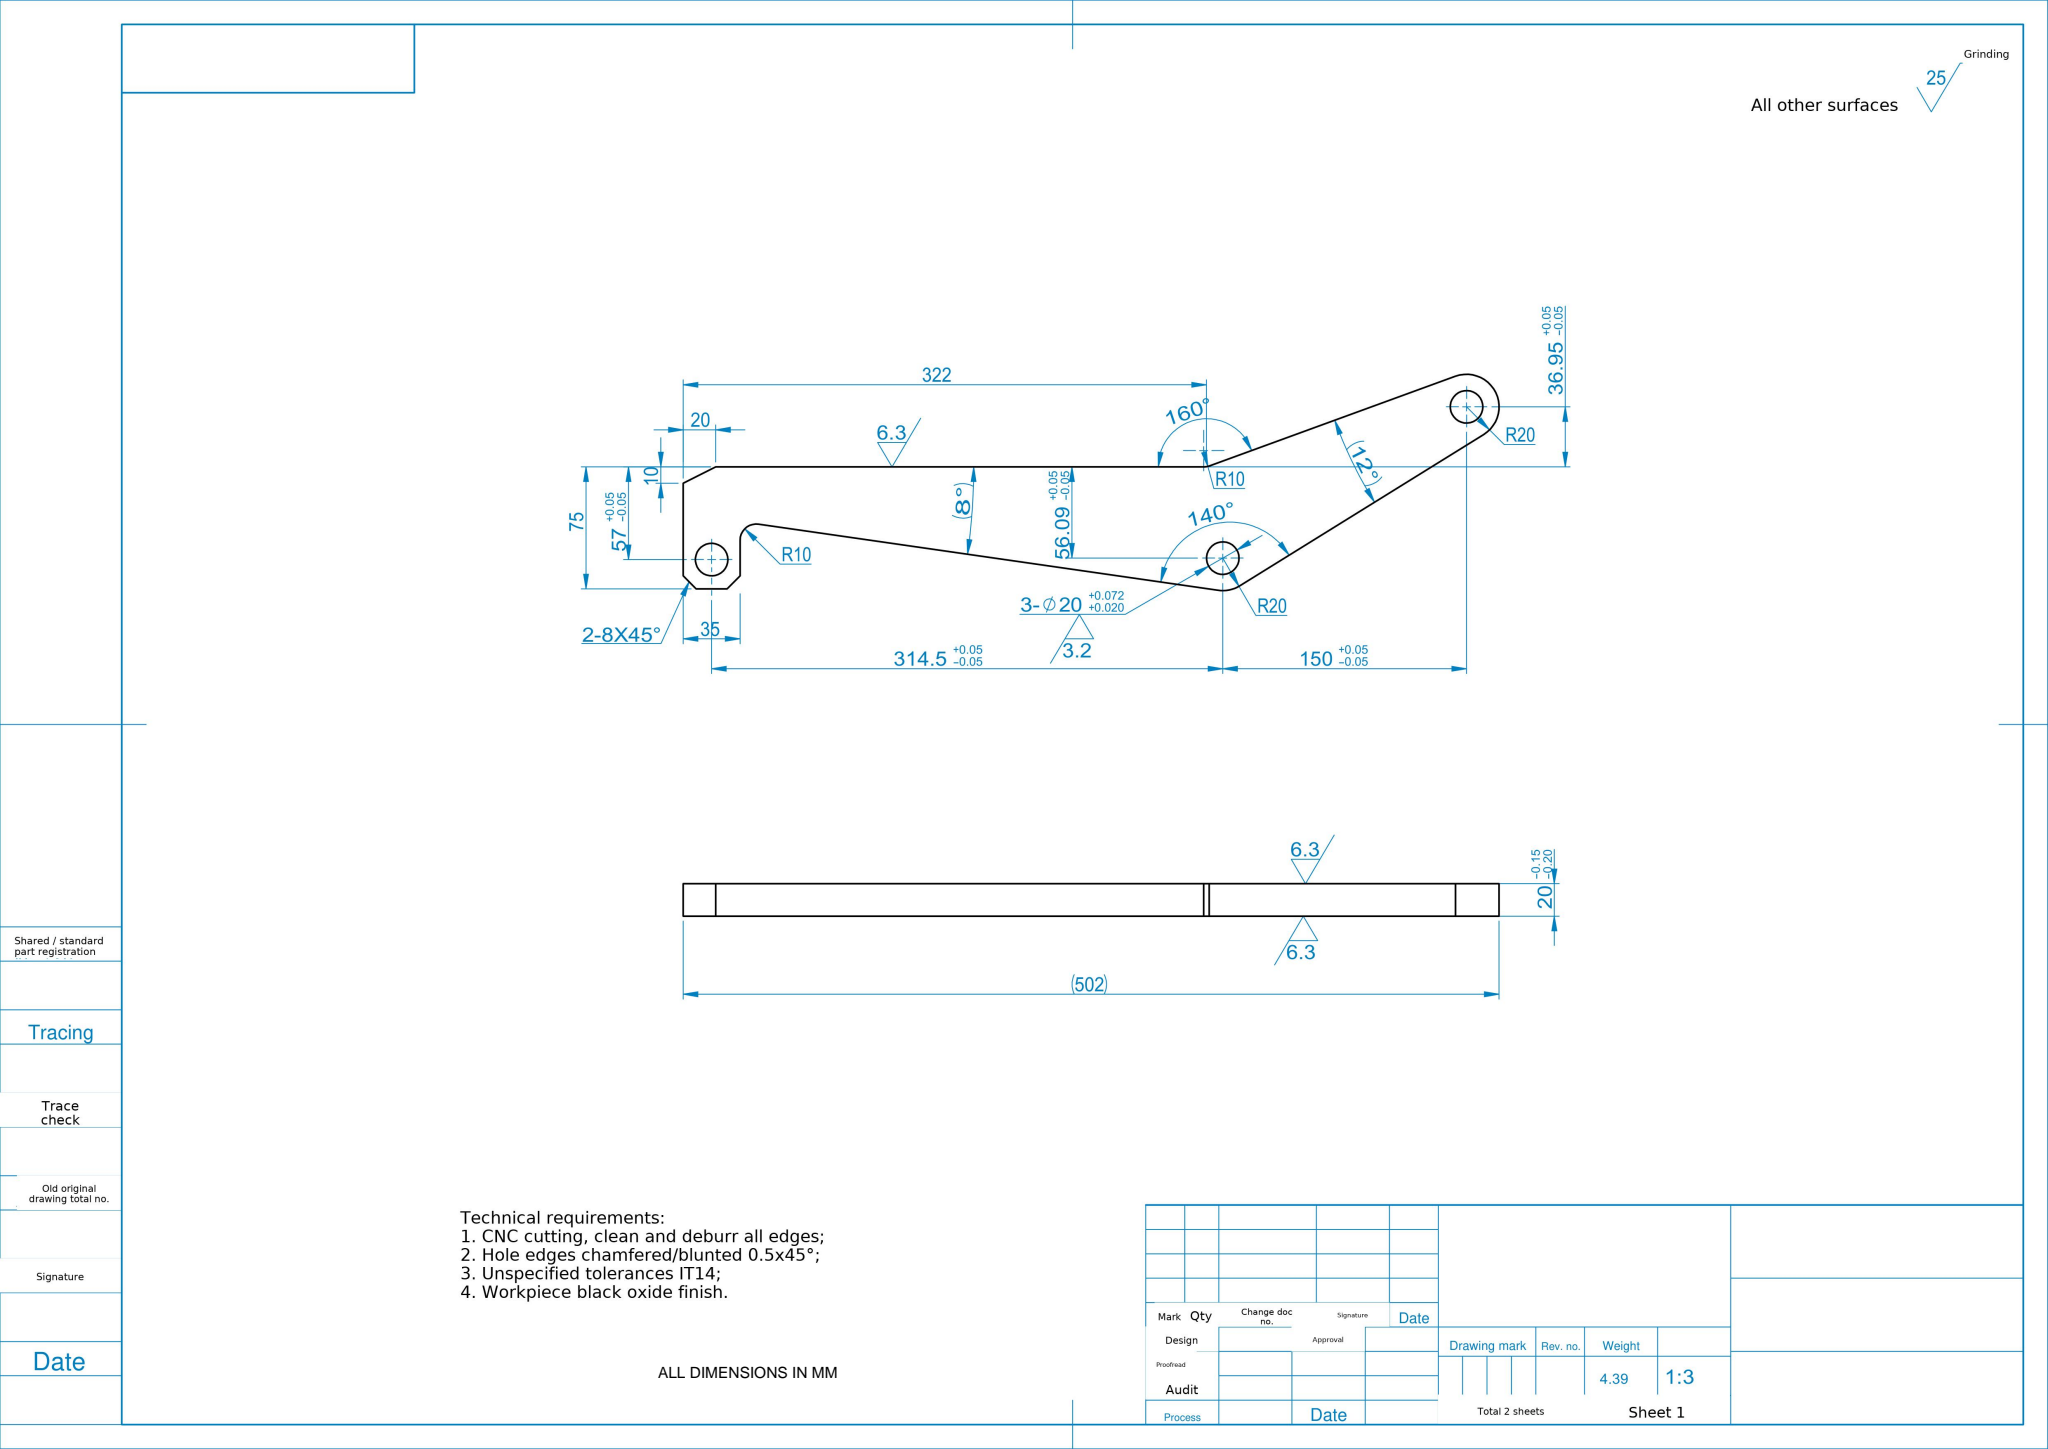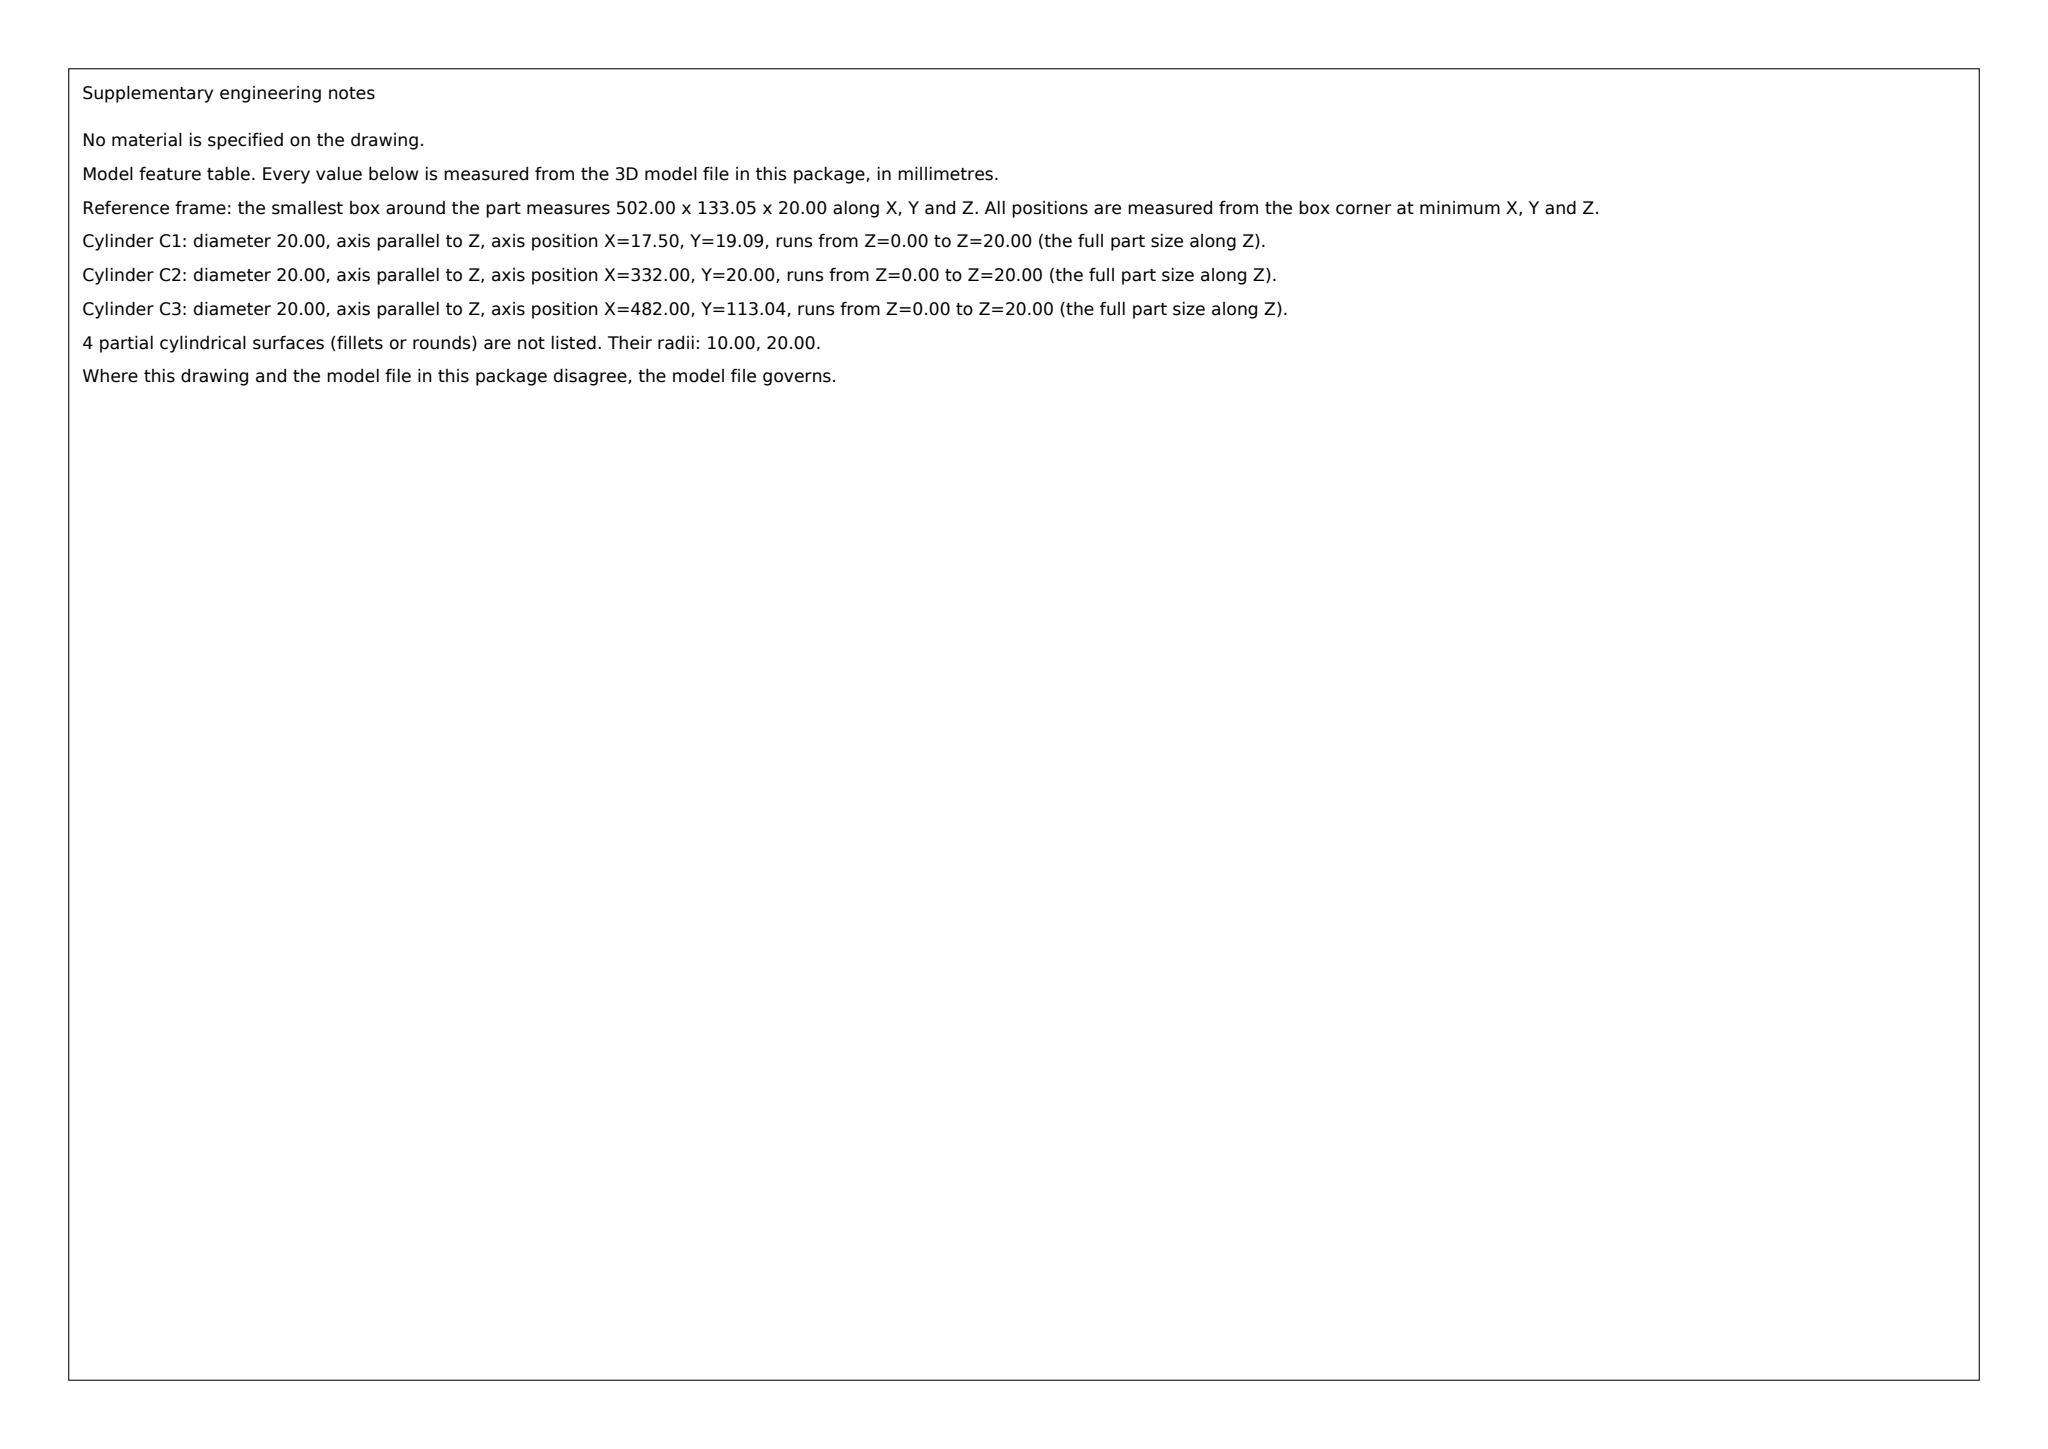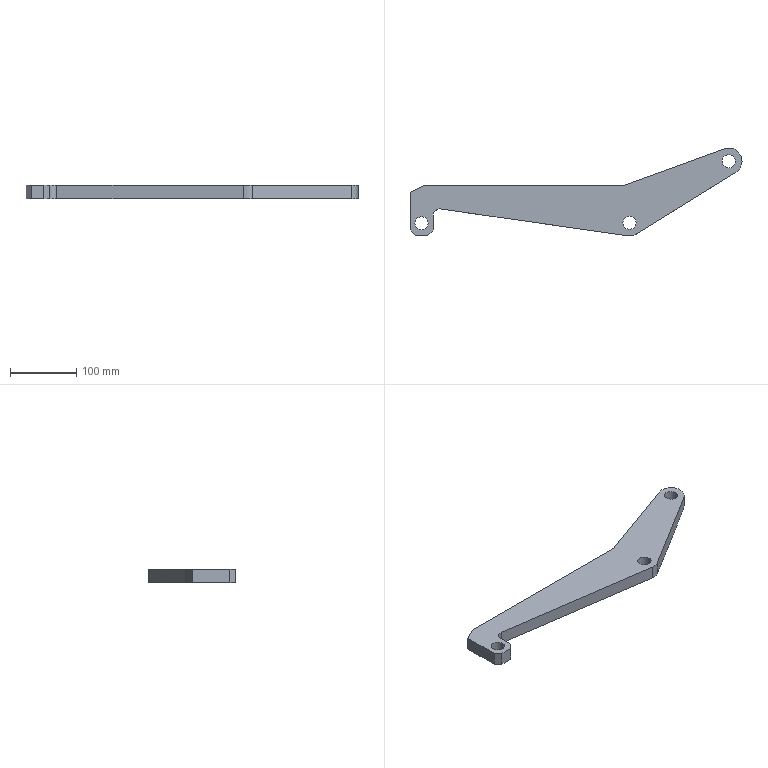Part | SolidWorks | mm | material Plain Carbon Steel | 1 solid | 22 faces | box 502 x 133.05 x 20 mm | volume 562252 mm3 | plane 12 | cylinder 10 | commonest cylinder face diameters 20 x8 40 x2
build123d program:
from build123d import *

# Parameters (mm, degrees)
BOSS_EXTRUDE1_DEPTH = 10
SKETCH2_R           = 10
CUT_EXTRUDE1_DEPTH  = 520.437
CHAMFER2_SIZE       = 8
CHAMFER3_SIZE       = 20
CHAMFER3_SIZE2      = 10
FILLET1_R           = 10
SKETCH5_R           = 10
CUT_EXTRUDE3_DEPTH  = 520.437
SKETCH7_R           = 10
CUT_EXTRUDE5_DEPTH  = 520.437
CUT_EXTRUDE6_DEPTH  = 520.437
FILLET2_R           = 10


with BuildPart() as part:
    # Sketch1 → Boss-Extrude1 (new, symmetric)
    with BuildSketch(Plane.XY):
        with BuildLine():
            Line((322, 75), (475.16, 130.746))
            ThreePointArc((475.16, 130.746), (499.99, 120.689), (492.542, 94.956))
            Line((492.542, 94.956), (342.542, 1.911))
            ThreePointArc((342.542, 1.911), (336.094, -0.6699), (329.151, -0.8894))
            Line((329.151, -0.8894), (45, 40))
            Line((45, 40), (35, 30))
            Line((35, 30), (35, 0))
            Line((35, 0), (0, 0))
            Line((0, 0), (0, 75))
            Line((0, 75), (322, 75))
        make_face()
    extrude(amount=BOSS_EXTRUDE1_DEPTH, both=True)

    # Sketch2 → Cut-Extrude1 (cut, through all)
    with BuildSketch(Plane.XY.offset(10)):
        with Locations((482, 111.952)):
            Circle(SKETCH2_R)
    extrude(amount=-CUT_EXTRUDE1_DEPTH, mode=Mode.SUBTRACT)

    # Chamfer2
    chamfer2_edges = [part.edges().sort_by_distance(p)[0] for p in [
        (35, 0, 0),
        (0, 0, 0),
    ]]
    chamfer(chamfer2_edges, length=CHAMFER2_SIZE)

    # Chamfer3
    chamfer3_edges = [part.edges().sort_by_distance(p)[0] for p in [
        (0, 75, 0),
    ]]
    chamfer3_side = [part.faces().sort_by_distance(p)[0] for p in [
        (161, 75, 0),
    ]]
    chamfer(chamfer3_edges, length=CHAMFER3_SIZE, length2=CHAMFER3_SIZE2, reference=chamfer3_side[0])

    # Fillet1
    fillet1_edges = [part.edges().sort_by_distance(p)[0] for p in [
        (322, 75, 0),
    ]]
    fillet(fillet1_edges, radius=FILLET1_R)

    # Sketch5 → Cut-Extrude3 (cut, through all)
    with BuildSketch(Plane.XY.offset(10)):
        with Locations((17.5, 18)):
            Circle(SKETCH5_R)
    extrude(amount=-CUT_EXTRUDE3_DEPTH, mode=Mode.SUBTRACT)

    # Sketch7 → Cut-Extrude5 (cut, through all)
    with BuildSketch(Plane.XY.offset(10)):
        with Locations((332, 18.907)):
            Circle(SKETCH7_R)
    extrude(amount=-CUT_EXTRUDE5_DEPTH, mode=Mode.SUBTRACT)

    # Sketch8 → Cut-Extrude6 (cut, through all)
    with BuildSketch(Plane.XY.offset(10)):
        Polygon((45, 40), (35, 30), (35, 41.439), align=None)
    extrude(amount=-CUT_EXTRUDE6_DEPTH, mode=Mode.SUBTRACT)

    # Fillet2
    fillet2_edges = [part.edges().sort_by_distance(p)[0] for p in [
        (35, 41.439, 0),
    ]]
    fillet(fillet2_edges, radius=FILLET2_R)


solid = part.part
STEP:
#1=CARTESIAN_POINT('',(322.,18.907,-10.));
#2=VERTEX_POINT('',#1);
#3=CARTESIAN_POINT('',(342.,18.907,-10.));
#4=VERTEX_POINT('',#3);
#5=CARTESIAN_POINT('',(332.,18.907,-10.));
#6=DIRECTION('',(0.,0.,1.));
#7=DIRECTION('',(1.,0.,0.));
#8=AXIS2_PLACEMENT_3D('',#5,#6,#7);
#9=CIRCLE('',#8,10.);
#10=EDGE_CURVE('',#2,#4,#9,.T.);
#11=ORIENTED_EDGE('',*,*,#10,.F.);
#12=CARTESIAN_POINT('',(322.,18.907,10.));
#13=VERTEX_POINT('',#12);
#14=CARTESIAN_POINT('',(322.,18.907,-10.));
#15=DIRECTION('',(0.,0.,1.));
#16=VECTOR('',#15,1000.);
#17=LINE('',#14,#16);
#18=EDGE_CURVE('',#2,#13,#17,.T.);
#19=ORIENTED_EDGE('',*,*,#18,.T.);
#20=CARTESIAN_POINT('',(342.,18.907,10.));
#21=VERTEX_POINT('',#20);
#22=CARTESIAN_POINT('',(332.,18.907,10.));
#23=DIRECTION('',(0.,0.,1.));
#24=DIRECTION('',(1.,0.,0.));
#25=AXIS2_PLACEMENT_3D('',#22,#23,#24);
#26=CIRCLE('',#25,10.);
#27=EDGE_CURVE('',#13,#21,#26,.T.);
#28=ORIENTED_EDGE('',*,*,#27,.T.);
#29=CARTESIAN_POINT('',(342.,18.907,-10.));
#30=DIRECTION('',(0.,0.,1.));
#31=VECTOR('',#30,1000.);
#32=LINE('',#29,#31);
#33=EDGE_CURVE('',#4,#21,#32,.T.);
#34=ORIENTED_EDGE('',*,*,#33,.F.);
#35=EDGE_LOOP('',(#11,#19,#28,#34));
#36=FACE_OUTER_BOUND('',#35,.T.);
#37=CARTESIAN_POINT('',(332.,18.907,-10.));
#38=DIRECTION('',(0.,0.,1.));
#39=DIRECTION('',(1.,0.,0.));
#40=AXIS2_PLACEMENT_3D('',#37,#38,#39);
#41=CYLINDRICAL_SURFACE('',#40,10.);
#42=ADVANCED_FACE('',(#36),#41,.F.);
#43=CARTESIAN_POINT('',(7.5,18.,-10.));
#44=VERTEX_POINT('',#43);
#45=CARTESIAN_POINT('',(27.5,18.,-10.));
#46=VERTEX_POINT('',#45);
#47=CARTESIAN_POINT('',(17.5,18.,-10.));
#48=DIRECTION('',(0.,0.,1.));
#49=DIRECTION('',(1.,0.,0.));
#50=AXIS2_PLACEMENT_3D('',#47,#48,#49);
#51=CIRCLE('',#50,10.);
#52=EDGE_CURVE('',#44,#46,#51,.T.);
#53=ORIENTED_EDGE('',*,*,#52,.F.);
#54=CARTESIAN_POINT('',(7.5,18.,10.));
#55=VERTEX_POINT('',#54);
#56=CARTESIAN_POINT('',(7.5,18.,-10.));
#57=DIRECTION('',(0.,0.,1.));
#58=VECTOR('',#57,1000.);
#59=LINE('',#56,#58);
#60=EDGE_CURVE('',#44,#55,#59,.T.);
#61=ORIENTED_EDGE('',*,*,#60,.T.);
#62=CARTESIAN_POINT('',(27.5,18.,10.));
#63=VERTEX_POINT('',#62);
#64=CARTESIAN_POINT('',(17.5,18.,10.));
#65=DIRECTION('',(0.,0.,1.));
#66=DIRECTION('',(1.,0.,0.));
#67=AXIS2_PLACEMENT_3D('',#64,#65,#66);
#68=CIRCLE('',#67,10.);
#69=EDGE_CURVE('',#55,#63,#68,.T.);
#70=ORIENTED_EDGE('',*,*,#69,.T.);
#71=CARTESIAN_POINT('',(27.5,18.,-10.));
#72=DIRECTION('',(0.,0.,1.));
#73=VECTOR('',#72,1000.);
#74=LINE('',#71,#73);
#75=EDGE_CURVE('',#46,#63,#74,.T.);
#76=ORIENTED_EDGE('',*,*,#75,.F.);
#77=EDGE_LOOP('',(#53,#61,#70,#76));
#78=FACE_OUTER_BOUND('',#77,.T.);
#79=CARTESIAN_POINT('',(17.5,18.,-10.));
#80=DIRECTION('',(0.,0.,1.));
#81=DIRECTION('',(1.,0.,0.));
#82=AXIS2_PLACEMENT_3D('',#79,#80,#81);
#83=CYLINDRICAL_SURFACE('',#82,10.);
#84=ADVANCED_FACE('',(#78),#83,.F.);
#85=CARTESIAN_POINT('',(472.,111.952,-10.));
#86=VERTEX_POINT('',#85);
#87=CARTESIAN_POINT('',(492.,111.952,-10.));
#88=VERTEX_POINT('',#87);
#89=CARTESIAN_POINT('',(482.,111.952,-10.));
#90=DIRECTION('',(0.,0.,1.));
#91=DIRECTION('',(1.,0.,0.));
#92=AXIS2_PLACEMENT_3D('',#89,#90,#91);
#93=CIRCLE('',#92,10.);
#94=EDGE_CURVE('',#86,#88,#93,.T.);
#95=ORIENTED_EDGE('',*,*,#94,.F.);
#96=CARTESIAN_POINT('',(472.,111.952,10.));
#97=VERTEX_POINT('',#96);
#98=CARTESIAN_POINT('',(472.,111.952,-10.));
#99=DIRECTION('',(0.,0.,1.));
#100=VECTOR('',#99,1000.);
#101=LINE('',#98,#100);
#102=EDGE_CURVE('',#86,#97,#101,.T.);
#103=ORIENTED_EDGE('',*,*,#102,.T.);
#104=CARTESIAN_POINT('',(492.,111.952,10.));
#105=VERTEX_POINT('',#104);
#106=CARTESIAN_POINT('',(482.,111.952,10.));
#107=DIRECTION('',(0.,0.,1.));
#108=DIRECTION('',(1.,0.,0.));
#109=AXIS2_PLACEMENT_3D('',#106,#107,#108);
#110=CIRCLE('',#109,10.);
#111=EDGE_CURVE('',#97,#105,#110,.T.);
#112=ORIENTED_EDGE('',*,*,#111,.T.);
#113=CARTESIAN_POINT('',(492.,111.952,-10.));
#114=DIRECTION('',(0.,0.,1.));
#115=VECTOR('',#114,1000.);
#116=LINE('',#113,#115);
#117=EDGE_CURVE('',#88,#105,#116,.T.);
#118=ORIENTED_EDGE('',*,*,#117,.F.);
#119=EDGE_LOOP('',(#95,#103,#112,#118));
#120=FACE_OUTER_BOUND('',#119,.T.);
#121=CARTESIAN_POINT('',(482.,111.952,-10.));
#122=DIRECTION('',(0.,0.,1.));
#123=DIRECTION('',(1.,0.,0.));
#124=AXIS2_PLACEMENT_3D('',#121,#122,#123);
#125=CYLINDRICAL_SURFACE('',#124,10.);
#126=ADVANCED_FACE('',(#120),#125,.F.);
#127=CARTESIAN_POINT('',(46.424,39.795,10.));
#128=VERTEX_POINT('',#127);
#129=CARTESIAN_POINT('',(329.151,-0.8894,10.));
#130=VERTEX_POINT('',#129);
#131=CARTESIAN_POINT('',(45.,40.,10.));
#132=DIRECTION('',(0.9898,-0.1424,0.));
#133=VECTOR('',#132,1000.);
#134=LINE('',#131,#133);
#135=EDGE_CURVE('',#128,#130,#134,.T.);
#136=ORIENTED_EDGE('',*,*,#135,.F.);
#137=CARTESIAN_POINT('',(46.424,39.795,-10.));
#138=VERTEX_POINT('',#137);
#139=CARTESIAN_POINT('',(46.424,39.795,-10.));
#140=DIRECTION('',(0.,0.,-1.));
#141=VECTOR('',#140,1000.);
#142=LINE('',#139,#141);
#143=EDGE_CURVE('',#128,#138,#142,.T.);
#144=ORIENTED_EDGE('',*,*,#143,.T.);
#145=CARTESIAN_POINT('',(329.151,-0.8894,-10.));
#146=VERTEX_POINT('',#145);
#147=CARTESIAN_POINT('',(45.,40.,-10.));
#148=DIRECTION('',(0.9898,-0.1424,0.));
#149=VECTOR('',#148,1000.);
#150=LINE('',#147,#149);
#151=EDGE_CURVE('',#138,#146,#150,.T.);
#152=ORIENTED_EDGE('',*,*,#151,.T.);
#153=CARTESIAN_POINT('',(329.151,-0.8894,10.));
#154=DIRECTION('',(0.,0.,-1.));
#155=VECTOR('',#154,1000.);
#156=LINE('',#153,#155);
#157=EDGE_CURVE('',#130,#146,#156,.T.);
#158=ORIENTED_EDGE('',*,*,#157,.F.);
#159=EDGE_LOOP('',(#136,#144,#152,#158));
#160=FACE_OUTER_BOUND('',#159,.T.);
#161=CARTESIAN_POINT('',(45.,40.,10.));
#162=DIRECTION('',(0.1424,0.9898,0.));
#163=DIRECTION('',(-0.9898,0.1424,0.));
#164=AXIS2_PLACEMENT_3D('',#161,#162,#163);
#165=PLANE('',#164);
#166=ADVANCED_FACE('',(#160),#165,.F.);
#167=CARTESIAN_POINT('',(342.542,1.911,-10.));
#168=VERTEX_POINT('',#167);
#169=CARTESIAN_POINT('',(332.,18.907,-10.));
#170=DIRECTION('',(0.,0.,1.));
#171=DIRECTION('',(1.,0.,0.));
#172=AXIS2_PLACEMENT_3D('',#169,#170,#171);
#173=CIRCLE('',#172,20.);
#174=EDGE_CURVE('',#146,#168,#173,.T.);
#175=ORIENTED_EDGE('',*,*,#174,.T.);
#176=CARTESIAN_POINT('',(342.542,1.911,10.));
#177=VERTEX_POINT('',#176);
#178=CARTESIAN_POINT('',(342.542,1.911,10.));
#179=DIRECTION('',(0.,0.,-1.));
#180=VECTOR('',#179,1000.);
#181=LINE('',#178,#180);
#182=EDGE_CURVE('',#177,#168,#181,.T.);
#183=ORIENTED_EDGE('',*,*,#182,.F.);
#184=CARTESIAN_POINT('',(332.,18.907,10.));
#185=DIRECTION('',(0.,0.,1.));
#186=DIRECTION('',(1.,0.,0.));
#187=AXIS2_PLACEMENT_3D('',#184,#185,#186);
#188=CIRCLE('',#187,20.);
#189=EDGE_CURVE('',#130,#177,#188,.T.);
#190=ORIENTED_EDGE('',*,*,#189,.F.);
#191=ORIENTED_EDGE('',*,*,#157,.T.);
#192=EDGE_LOOP('',(#175,#183,#190,#191));
#193=FACE_OUTER_BOUND('',#192,.T.);
#194=CARTESIAN_POINT('',(332.,18.907,10.));
#195=DIRECTION('',(0.,0.,-1.));
#196=DIRECTION('',(-1.,0.,0.));
#197=AXIS2_PLACEMENT_3D('',#194,#195,#196);
#198=CYLINDRICAL_SURFACE('',#197,20.);
#199=ADVANCED_FACE('',(#193),#198,.T.);
#200=CARTESIAN_POINT('',(492.542,94.956,-10.));
#201=VERTEX_POINT('',#200);
#202=CARTESIAN_POINT('',(342.542,1.911,-10.));
#203=DIRECTION('',(0.8498,0.5271,0.));
#204=VECTOR('',#203,1000.);
#205=LINE('',#202,#204);
#206=EDGE_CURVE('',#168,#201,#205,.T.);
#207=ORIENTED_EDGE('',*,*,#206,.T.);
#208=CARTESIAN_POINT('',(492.542,94.956,10.));
#209=VERTEX_POINT('',#208);
#210=CARTESIAN_POINT('',(492.542,94.956,10.));
#211=DIRECTION('',(0.,0.,-1.));
#212=VECTOR('',#211,1000.);
#213=LINE('',#210,#212);
#214=EDGE_CURVE('',#209,#201,#213,.T.);
#215=ORIENTED_EDGE('',*,*,#214,.F.);
#216=CARTESIAN_POINT('',(342.542,1.911,10.));
#217=DIRECTION('',(0.8498,0.5271,0.));
#218=VECTOR('',#217,1000.);
#219=LINE('',#216,#218);
#220=EDGE_CURVE('',#177,#209,#219,.T.);
#221=ORIENTED_EDGE('',*,*,#220,.F.);
#222=ORIENTED_EDGE('',*,*,#182,.T.);
#223=EDGE_LOOP('',(#207,#215,#221,#222));
#224=FACE_OUTER_BOUND('',#223,.T.);
#225=CARTESIAN_POINT('',(342.542,1.911,10.));
#226=DIRECTION('',(-0.5271,0.8498,0.));
#227=DIRECTION('',(-0.8498,-0.5271,0.));
#228=AXIS2_PLACEMENT_3D('',#225,#226,#227);
#229=PLANE('',#228);
#230=ADVANCED_FACE('',(#224),#229,.F.);
#231=CARTESIAN_POINT('',(475.16,130.746,-10.));
#232=VERTEX_POINT('',#231);
#233=CARTESIAN_POINT('',(482.,111.952,-10.));
#234=DIRECTION('',(0.,0.,1.));
#235=DIRECTION('',(1.,0.,0.));
#236=AXIS2_PLACEMENT_3D('',#233,#234,#235);
#237=CIRCLE('',#236,20.);
#238=EDGE_CURVE('',#201,#232,#237,.T.);
#239=ORIENTED_EDGE('',*,*,#238,.T.);
#240=CARTESIAN_POINT('',(475.16,130.746,10.));
#241=VERTEX_POINT('',#240);
#242=CARTESIAN_POINT('',(475.16,130.746,10.));
#243=DIRECTION('',(0.,0.,-1.));
#244=VECTOR('',#243,1000.);
#245=LINE('',#242,#244);
#246=EDGE_CURVE('',#241,#232,#245,.T.);
#247=ORIENTED_EDGE('',*,*,#246,.F.);
#248=CARTESIAN_POINT('',(482.,111.952,10.));
#249=DIRECTION('',(0.,0.,1.));
#250=DIRECTION('',(1.,0.,0.));
#251=AXIS2_PLACEMENT_3D('',#248,#249,#250);
#252=CIRCLE('',#251,20.);
#253=EDGE_CURVE('',#209,#241,#252,.T.);
#254=ORIENTED_EDGE('',*,*,#253,.F.);
#255=ORIENTED_EDGE('',*,*,#214,.T.);
#256=EDGE_LOOP('',(#239,#247,#254,#255));
#257=FACE_OUTER_BOUND('',#256,.T.);
#258=CARTESIAN_POINT('',(482.,111.952,10.));
#259=DIRECTION('',(0.,0.,-1.));
#260=DIRECTION('',(-1.,0.,0.));
#261=AXIS2_PLACEMENT_3D('',#258,#259,#260);
#262=CYLINDRICAL_SURFACE('',#261,20.);
#263=ADVANCED_FACE('',(#257),#262,.T.);
#264=CARTESIAN_POINT('',(323.657,75.603,-10.));
#265=VERTEX_POINT('',#264);
#266=CARTESIAN_POINT('',(322.,75.,-10.));
#267=DIRECTION('',(-0.9397,-0.342,0.));
#268=VECTOR('',#267,1000.);
#269=LINE('',#266,#268);
#270=EDGE_CURVE('',#232,#265,#269,.T.);
#271=ORIENTED_EDGE('',*,*,#270,.T.);
#272=CARTESIAN_POINT('',(323.657,75.603,10.));
#273=VERTEX_POINT('',#272);
#274=CARTESIAN_POINT('',(323.657,75.603,10.));
#275=DIRECTION('',(0.,0.,1.));
#276=VECTOR('',#275,1000.);
#277=LINE('',#274,#276);
#278=EDGE_CURVE('',#265,#273,#277,.T.);
#279=ORIENTED_EDGE('',*,*,#278,.T.);
#280=CARTESIAN_POINT('',(322.,75.,10.));
#281=DIRECTION('',(-0.9397,-0.342,0.));
#282=VECTOR('',#281,1000.);
#283=LINE('',#280,#282);
#284=EDGE_CURVE('',#241,#273,#283,.T.);
#285=ORIENTED_EDGE('',*,*,#284,.F.);
#286=ORIENTED_EDGE('',*,*,#246,.T.);
#287=EDGE_LOOP('',(#271,#279,#285,#286));
#288=FACE_OUTER_BOUND('',#287,.T.);
#289=CARTESIAN_POINT('',(322.,75.,10.));
#290=DIRECTION('',(0.342,-0.9397,0.));
#291=DIRECTION('',(0.9397,0.342,0.));
#292=AXIS2_PLACEMENT_3D('',#289,#290,#291);
#293=PLANE('',#292);
#294=ADVANCED_FACE('',(#288),#293,.F.);
#295=CARTESIAN_POINT('',(320.237,75.,10.));
#296=VERTEX_POINT('',#295);
#297=CARTESIAN_POINT('',(20.,75.,10.));
#298=VERTEX_POINT('',#297);
#299=CARTESIAN_POINT('',(0.,75.,10.));
#300=DIRECTION('',(-1.,-0.,0.));
#301=VECTOR('',#300,1000.);
#302=LINE('',#299,#301);
#303=EDGE_CURVE('',#296,#298,#302,.T.);
#304=ORIENTED_EDGE('',*,*,#303,.F.);
#305=CARTESIAN_POINT('',(320.237,75.,-10.));
#306=VERTEX_POINT('',#305);
#307=CARTESIAN_POINT('',(320.237,75.,-10.));
#308=DIRECTION('',(0.,0.,-1.));
#309=VECTOR('',#308,1000.);
#310=LINE('',#307,#309);
#311=EDGE_CURVE('',#296,#306,#310,.T.);
#312=ORIENTED_EDGE('',*,*,#311,.T.);
#313=CARTESIAN_POINT('',(20.,75.,-10.));
#314=VERTEX_POINT('',#313);
#315=CARTESIAN_POINT('',(0.,75.,-10.));
#316=DIRECTION('',(-1.,-0.,0.));
#317=VECTOR('',#316,1000.);
#318=LINE('',#315,#317);
#319=EDGE_CURVE('',#306,#314,#318,.T.);
#320=ORIENTED_EDGE('',*,*,#319,.T.);
#321=CARTESIAN_POINT('',(20.,75.,10.));
#322=DIRECTION('',(0.,0.,1.));
#323=VECTOR('',#322,1000.);
#324=LINE('',#321,#323);
#325=EDGE_CURVE('',#314,#298,#324,.T.);
#326=ORIENTED_EDGE('',*,*,#325,.T.);
#327=EDGE_LOOP('',(#304,#312,#320,#326));
#328=FACE_OUTER_BOUND('',#327,.T.);
#329=CARTESIAN_POINT('',(0.,75.,10.));
#330=DIRECTION('',(0.,-1.,0.));
#331=DIRECTION('',(1.,0.,0.));
#332=AXIS2_PLACEMENT_3D('',#329,#330,#331);
#333=PLANE('',#332);
#334=ADVANCED_FACE('',(#328),#333,.F.);
#335=CARTESIAN_POINT('',(-0.,65.,10.));
#336=VERTEX_POINT('',#335);
#337=CARTESIAN_POINT('',(-0.,8.,10.));
#338=VERTEX_POINT('',#337);
#339=CARTESIAN_POINT('',(0.,0.,10.));
#340=DIRECTION('',(0.,-1.,0.));
#341=VECTOR('',#340,1000.);
#342=LINE('',#339,#341);
#343=EDGE_CURVE('',#336,#338,#342,.T.);
#344=ORIENTED_EDGE('',*,*,#343,.F.);
#345=CARTESIAN_POINT('',(-0.,65.,-10.));
#346=VERTEX_POINT('',#345);
#347=CARTESIAN_POINT('',(0.,65.,10.));
#348=DIRECTION('',(0.,0.,-1.));
#349=VECTOR('',#348,1000.);
#350=LINE('',#347,#349);
#351=EDGE_CURVE('',#336,#346,#350,.T.);
#352=ORIENTED_EDGE('',*,*,#351,.T.);
#353=CARTESIAN_POINT('',(0.,8.,-10.));
#354=VERTEX_POINT('',#353);
#355=CARTESIAN_POINT('',(0.,0.,-10.));
#356=DIRECTION('',(0.,-1.,0.));
#357=VECTOR('',#356,1000.);
#358=LINE('',#355,#357);
#359=EDGE_CURVE('',#346,#354,#358,.T.);
#360=ORIENTED_EDGE('',*,*,#359,.T.);
#361=CARTESIAN_POINT('',(0.,8.,10.));
#362=DIRECTION('',(0.,0.,1.));
#363=VECTOR('',#362,1000.);
#364=LINE('',#361,#363);
#365=EDGE_CURVE('',#354,#338,#364,.T.);
#366=ORIENTED_EDGE('',*,*,#365,.T.);
#367=EDGE_LOOP('',(#344,#352,#360,#366));
#368=FACE_OUTER_BOUND('',#367,.T.);
#369=CARTESIAN_POINT('',(0.,0.,10.));
#370=DIRECTION('',(1.,0.,0.));
#371=DIRECTION('',(0.,0.,-1.));
#372=AXIS2_PLACEMENT_3D('',#369,#370,#371);
#373=PLANE('',#372);
#374=ADVANCED_FACE('',(#368),#373,.F.);
#375=CARTESIAN_POINT('',(8.,-0.,-10.));
#376=VERTEX_POINT('',#375);
#377=CARTESIAN_POINT('',(27.,0.,-10.));
#378=VERTEX_POINT('',#377);
#379=CARTESIAN_POINT('',(35.,0.,-10.));
#380=DIRECTION('',(1.,0.,0.));
#381=VECTOR('',#380,1000.);
#382=LINE('',#379,#381);
#383=EDGE_CURVE('',#376,#378,#382,.T.);
#384=ORIENTED_EDGE('',*,*,#383,.T.);
#385=CARTESIAN_POINT('',(27.,-0.,10.));
#386=VERTEX_POINT('',#385);
#387=CARTESIAN_POINT('',(27.,0.,10.));
#388=DIRECTION('',(0.,0.,1.));
#389=VECTOR('',#388,1000.);
#390=LINE('',#387,#389);
#391=EDGE_CURVE('',#378,#386,#390,.T.);
#392=ORIENTED_EDGE('',*,*,#391,.T.);
#393=CARTESIAN_POINT('',(8.,0.,10.));
#394=VERTEX_POINT('',#393);
#395=CARTESIAN_POINT('',(35.,0.,10.));
#396=DIRECTION('',(1.,0.,0.));
#397=VECTOR('',#396,1000.);
#398=LINE('',#395,#397);
#399=EDGE_CURVE('',#394,#386,#398,.T.);
#400=ORIENTED_EDGE('',*,*,#399,.F.);
#401=CARTESIAN_POINT('',(8.,0.,10.));
#402=DIRECTION('',(0.,0.,-1.));
#403=VECTOR('',#402,1000.);
#404=LINE('',#401,#403);
#405=EDGE_CURVE('',#394,#376,#404,.T.);
#406=ORIENTED_EDGE('',*,*,#405,.T.);
#407=EDGE_LOOP('',(#384,#392,#400,#406));
#408=FACE_OUTER_BOUND('',#407,.T.);
#409=CARTESIAN_POINT('',(35.,0.,10.));
#410=DIRECTION('',(-0.,1.,0.));
#411=DIRECTION('',(-1.,-0.,0.));
#412=AXIS2_PLACEMENT_3D('',#409,#410,#411);
#413=PLANE('',#412);
#414=ADVANCED_FACE('',(#408),#413,.F.);
#415=CARTESIAN_POINT('',(35.,8.,-10.));
#416=VERTEX_POINT('',#415);
#417=CARTESIAN_POINT('',(35.,29.897,-10.));
#418=VERTEX_POINT('',#417);
#419=CARTESIAN_POINT('',(35.,30.,-10.));
#420=DIRECTION('',(0.,1.,0.));
#421=VECTOR('',#420,1000.);
#422=LINE('',#419,#421);
#423=EDGE_CURVE('',#416,#418,#422,.T.);
#424=ORIENTED_EDGE('',*,*,#423,.T.);
#425=CARTESIAN_POINT('',(35.,29.897,10.));
#426=VERTEX_POINT('',#425);
#427=CARTESIAN_POINT('',(35.,29.897,10.));
#428=DIRECTION('',(0.,0.,1.));
#429=VECTOR('',#428,1000.);
#430=LINE('',#427,#429);
#431=EDGE_CURVE('',#418,#426,#430,.T.);
#432=ORIENTED_EDGE('',*,*,#431,.T.);
#433=CARTESIAN_POINT('',(35.,8.,10.));
#434=VERTEX_POINT('',#433);
#435=CARTESIAN_POINT('',(35.,30.,10.));
#436=DIRECTION('',(0.,1.,0.));
#437=VECTOR('',#436,1000.);
#438=LINE('',#435,#437);
#439=EDGE_CURVE('',#434,#426,#438,.T.);
#440=ORIENTED_EDGE('',*,*,#439,.F.);
#441=CARTESIAN_POINT('',(35.,8.,10.));
#442=DIRECTION('',(0.,0.,-1.));
#443=VECTOR('',#442,1000.);
#444=LINE('',#441,#443);
#445=EDGE_CURVE('',#434,#416,#444,.T.);
#446=ORIENTED_EDGE('',*,*,#445,.T.);
#447=EDGE_LOOP('',(#424,#432,#440,#446));
#448=FACE_OUTER_BOUND('',#447,.T.);
#449=CARTESIAN_POINT('',(35.,30.,10.));
#450=DIRECTION('',(-1.,0.,0.));
#451=DIRECTION('',(0.,0.,1.));
#452=AXIS2_PLACEMENT_3D('',#449,#450,#451);
#453=PLANE('',#452);
#454=ADVANCED_FACE('',(#448),#453,.F.);
#455=ORIENTED_EDGE('',*,*,#439,.T.);
#456=CARTESIAN_POINT('',(45.,29.897,10.));
#457=DIRECTION('',(0.,0.,-1.));
#458=DIRECTION('',(1.,0.,0.));
#459=AXIS2_PLACEMENT_3D('',#456,#457,#458);
#460=CIRCLE('',#459,10.);
#461=EDGE_CURVE('',#426,#128,#460,.T.);
#462=ORIENTED_EDGE('',*,*,#461,.T.);
#463=ORIENTED_EDGE('',*,*,#135,.T.);
#464=ORIENTED_EDGE('',*,*,#189,.T.);
#465=ORIENTED_EDGE('',*,*,#220,.T.);
#466=ORIENTED_EDGE('',*,*,#253,.T.);
#467=ORIENTED_EDGE('',*,*,#284,.T.);
#468=CARTESIAN_POINT('',(320.237,85.,10.));
#469=DIRECTION('',(0.,0.,-1.));
#470=DIRECTION('',(1.,0.,0.));
#471=AXIS2_PLACEMENT_3D('',#468,#469,#470);
#472=CIRCLE('',#471,10.);
#473=EDGE_CURVE('',#273,#296,#472,.T.);
#474=ORIENTED_EDGE('',*,*,#473,.T.);
#475=ORIENTED_EDGE('',*,*,#303,.T.);
#476=CARTESIAN_POINT('',(247.163,188.581,10.));
#477=DIRECTION('',(-0.8944,-0.4472,0.));
#478=VECTOR('',#477,1000.);
#479=LINE('',#476,#478);
#480=EDGE_CURVE('',#298,#336,#479,.T.);
#481=ORIENTED_EDGE('',*,*,#480,.T.);
#482=ORIENTED_EDGE('',*,*,#343,.T.);
#483=CARTESIAN_POINT('',(160.547,-152.547,10.));
#484=DIRECTION('',(0.7071,-0.7071,0.));
#485=VECTOR('',#484,1000.);
#486=LINE('',#483,#485);
#487=EDGE_CURVE('',#338,#394,#486,.T.);
#488=ORIENTED_EDGE('',*,*,#487,.T.);
#489=ORIENTED_EDGE('',*,*,#399,.T.);
#490=CARTESIAN_POINT('',(188.953,161.953,10.));
#491=DIRECTION('',(0.7071,0.7071,0.));
#492=VECTOR('',#491,1000.);
#493=LINE('',#490,#492);
#494=EDGE_CURVE('',#386,#434,#493,.T.);
#495=ORIENTED_EDGE('',*,*,#494,.T.);
#496=EDGE_LOOP('',(#455,#462,#463,#464,#465,#466,#467,#474,#475,#481,#482,#488,#489,#495));
#497=FACE_OUTER_BOUND('',#496,.T.);
#498=CARTESIAN_POINT('',(332.,18.907,10.));
#499=DIRECTION('',(0.,0.,1.));
#500=DIRECTION('',(1.,0.,0.));
#501=AXIS2_PLACEMENT_3D('',#498,#499,#500);
#502=CIRCLE('',#501,10.);
#503=EDGE_CURVE('',#21,#13,#502,.T.);
#504=ORIENTED_EDGE('',*,*,#503,.F.);
#505=ORIENTED_EDGE('',*,*,#27,.F.);
#506=EDGE_LOOP('',(#504,#505));
#507=FACE_BOUND('',#506,.T.);
#508=CARTESIAN_POINT('',(17.5,18.,10.));
#509=DIRECTION('',(0.,0.,1.));
#510=DIRECTION('',(1.,0.,0.));
#511=AXIS2_PLACEMENT_3D('',#508,#509,#510);
#512=CIRCLE('',#511,10.);
#513=EDGE_CURVE('',#63,#55,#512,.T.);
#514=ORIENTED_EDGE('',*,*,#513,.F.);
#515=ORIENTED_EDGE('',*,*,#69,.F.);
#516=EDGE_LOOP('',(#514,#515));
#517=FACE_BOUND('',#516,.T.);
#518=CARTESIAN_POINT('',(482.,111.952,10.));
#519=DIRECTION('',(0.,0.,1.));
#520=DIRECTION('',(1.,0.,0.));
#521=AXIS2_PLACEMENT_3D('',#518,#519,#520);
#522=CIRCLE('',#521,10.);
#523=EDGE_CURVE('',#105,#97,#522,.T.);
#524=ORIENTED_EDGE('',*,*,#523,.F.);
#525=ORIENTED_EDGE('',*,*,#111,.F.);
#526=EDGE_LOOP('',(#524,#525));
#527=FACE_BOUND('',#526,.T.);
#528=CARTESIAN_POINT('',(332.,18.907,10.));
#529=DIRECTION('',(0.,0.,1.));
#530=DIRECTION('',(1.,0.,0.));
#531=AXIS2_PLACEMENT_3D('',#528,#529,#530);
#532=PLANE('',#531);
#533=ADVANCED_FACE('',(#497,#507,#517,#527),#532,.T.);
#534=CARTESIAN_POINT('',(332.,18.907,-10.));
#535=DIRECTION('',(0.,0.,1.));
#536=DIRECTION('',(1.,0.,0.));
#537=AXIS2_PLACEMENT_3D('',#534,#535,#536);
#538=CIRCLE('',#537,10.);
#539=EDGE_CURVE('',#4,#2,#538,.T.);
#540=ORIENTED_EDGE('',*,*,#539,.T.);
#541=ORIENTED_EDGE('',*,*,#10,.T.);
#542=EDGE_LOOP('',(#540,#541));
#543=FACE_BOUND('',#542,.T.);
#544=CARTESIAN_POINT('',(17.5,18.,-10.));
#545=DIRECTION('',(0.,0.,1.));
#546=DIRECTION('',(1.,0.,0.));
#547=AXIS2_PLACEMENT_3D('',#544,#545,#546);
#548=CIRCLE('',#547,10.);
#549=EDGE_CURVE('',#46,#44,#548,.T.);
#550=ORIENTED_EDGE('',*,*,#549,.T.);
#551=ORIENTED_EDGE('',*,*,#52,.T.);
#552=EDGE_LOOP('',(#550,#551));
#553=FACE_BOUND('',#552,.T.);
#554=CARTESIAN_POINT('',(482.,111.952,-10.));
#555=DIRECTION('',(0.,0.,1.));
#556=DIRECTION('',(1.,0.,0.));
#557=AXIS2_PLACEMENT_3D('',#554,#555,#556);
#558=CIRCLE('',#557,10.);
#559=EDGE_CURVE('',#88,#86,#558,.T.);
#560=ORIENTED_EDGE('',*,*,#559,.T.);
#561=ORIENTED_EDGE('',*,*,#94,.T.);
#562=EDGE_LOOP('',(#560,#561));
#563=FACE_BOUND('',#562,.T.);
#564=ORIENTED_EDGE('',*,*,#151,.F.);
#565=CARTESIAN_POINT('',(45.,29.897,-10.));
#566=DIRECTION('',(0.,0.,1.));
#567=DIRECTION('',(1.,0.,0.));
#568=AXIS2_PLACEMENT_3D('',#565,#566,#567);
#569=CIRCLE('',#568,10.);
#570=EDGE_CURVE('',#138,#418,#569,.T.);
#571=ORIENTED_EDGE('',*,*,#570,.T.);
#572=ORIENTED_EDGE('',*,*,#423,.F.);
#573=CARTESIAN_POINT('',(35.,8.,-10.));
#574=DIRECTION('',(-0.7071,-0.7071,0.));
#575=VECTOR('',#574,1000.);
#576=LINE('',#573,#575);
#577=EDGE_CURVE('',#416,#378,#576,.T.);
#578=ORIENTED_EDGE('',*,*,#577,.T.);
#579=ORIENTED_EDGE('',*,*,#383,.F.);
#580=CARTESIAN_POINT('',(8.,0.,-10.));
#581=DIRECTION('',(-0.7071,0.7071,0.));
#582=VECTOR('',#581,1000.);
#583=LINE('',#580,#582);
#584=EDGE_CURVE('',#376,#354,#583,.T.);
#585=ORIENTED_EDGE('',*,*,#584,.T.);
#586=ORIENTED_EDGE('',*,*,#359,.F.);
#587=CARTESIAN_POINT('',(0.,65.,-10.));
#588=DIRECTION('',(0.8944,0.4472,0.));
#589=VECTOR('',#588,1000.);
#590=LINE('',#587,#589);
#591=EDGE_CURVE('',#346,#314,#590,.T.);
#592=ORIENTED_EDGE('',*,*,#591,.T.);
#593=ORIENTED_EDGE('',*,*,#319,.F.);
#594=CARTESIAN_POINT('',(320.237,85.,-10.));
#595=DIRECTION('',(0.,0.,1.));
#596=DIRECTION('',(1.,0.,0.));
#597=AXIS2_PLACEMENT_3D('',#594,#595,#596);
#598=CIRCLE('',#597,10.);
#599=EDGE_CURVE('',#306,#265,#598,.T.);
#600=ORIENTED_EDGE('',*,*,#599,.T.);
#601=ORIENTED_EDGE('',*,*,#270,.F.);
#602=ORIENTED_EDGE('',*,*,#238,.F.);
#603=ORIENTED_EDGE('',*,*,#206,.F.);
#604=ORIENTED_EDGE('',*,*,#174,.F.);
#605=EDGE_LOOP('',(#564,#571,#572,#578,#579,#585,#586,#592,#593,#600,#601,#602,#603,#604));
#606=FACE_OUTER_BOUND('',#605,.T.);
#607=CARTESIAN_POINT('',(332.,18.907,-10.));
#608=DIRECTION('',(0.,0.,1.));
#609=DIRECTION('',(1.,0.,0.));
#610=AXIS2_PLACEMENT_3D('',#607,#608,#609);
#611=PLANE('',#610);
#612=ADVANCED_FACE('',(#543,#553,#563,#606),#611,.F.);
#613=ORIENTED_EDGE('',*,*,#102,.F.);
#614=ORIENTED_EDGE('',*,*,#559,.F.);
#615=ORIENTED_EDGE('',*,*,#117,.T.);
#616=ORIENTED_EDGE('',*,*,#523,.T.);
#617=EDGE_LOOP('',(#613,#614,#615,#616));
#618=FACE_OUTER_BOUND('',#617,.T.);
#619=CARTESIAN_POINT('',(482.,111.952,-10.));
#620=DIRECTION('',(0.,0.,1.));
#621=DIRECTION('',(1.,0.,0.));
#622=AXIS2_PLACEMENT_3D('',#619,#620,#621);
#623=CYLINDRICAL_SURFACE('',#622,10.);
#624=ADVANCED_FACE('',(#618),#623,.F.);
#625=ORIENTED_EDGE('',*,*,#494,.F.);
#626=ORIENTED_EDGE('',*,*,#391,.F.);
#627=ORIENTED_EDGE('',*,*,#577,.F.);
#628=ORIENTED_EDGE('',*,*,#445,.F.);
#629=EDGE_LOOP('',(#625,#626,#627,#628));
#630=FACE_OUTER_BOUND('',#629,.T.);
#631=CARTESIAN_POINT('',(35.,8.,10.));
#632=DIRECTION('',(-0.7071,0.7071,0.));
#633=DIRECTION('',(0.,0.,-1.));
#634=AXIS2_PLACEMENT_3D('',#631,#632,#633);
#635=PLANE('',#634);
#636=ADVANCED_FACE('',(#630),#635,.F.);
#637=ORIENTED_EDGE('',*,*,#487,.F.);
#638=ORIENTED_EDGE('',*,*,#365,.F.);
#639=ORIENTED_EDGE('',*,*,#584,.F.);
#640=ORIENTED_EDGE('',*,*,#405,.F.);
#641=EDGE_LOOP('',(#637,#638,#639,#640));
#642=FACE_OUTER_BOUND('',#641,.T.);
#643=CARTESIAN_POINT('',(8.,0.,10.));
#644=DIRECTION('',(0.7071,0.7071,0.));
#645=DIRECTION('',(0.,0.,-1.));
#646=AXIS2_PLACEMENT_3D('',#643,#644,#645);
#647=PLANE('',#646);
#648=ADVANCED_FACE('',(#642),#647,.F.);
#649=ORIENTED_EDGE('',*,*,#480,.F.);
#650=ORIENTED_EDGE('',*,*,#325,.F.);
#651=ORIENTED_EDGE('',*,*,#591,.F.);
#652=ORIENTED_EDGE('',*,*,#351,.F.);
#653=EDGE_LOOP('',(#649,#650,#651,#652));
#654=FACE_OUTER_BOUND('',#653,.T.);
#655=CARTESIAN_POINT('',(0.,65.,10.));
#656=DIRECTION('',(0.4472,-0.8944,0.));
#657=DIRECTION('',(0.,0.,-1.));
#658=AXIS2_PLACEMENT_3D('',#655,#656,#657);
#659=PLANE('',#658);
#660=ADVANCED_FACE('',(#654),#659,.F.);
#661=ORIENTED_EDGE('',*,*,#473,.F.);
#662=ORIENTED_EDGE('',*,*,#278,.F.);
#663=ORIENTED_EDGE('',*,*,#599,.F.);
#664=ORIENTED_EDGE('',*,*,#311,.F.);
#665=EDGE_LOOP('',(#661,#662,#663,#664));
#666=FACE_OUTER_BOUND('',#665,.T.);
#667=CARTESIAN_POINT('',(320.237,85.,10.));
#668=DIRECTION('',(0.,0.,1.));
#669=DIRECTION('',(1.,0.,0.));
#670=AXIS2_PLACEMENT_3D('',#667,#668,#669);
#671=CYLINDRICAL_SURFACE('',#670,10.);
#672=ADVANCED_FACE('',(#666),#671,.F.);
#673=ORIENTED_EDGE('',*,*,#60,.F.);
#674=ORIENTED_EDGE('',*,*,#549,.F.);
#675=ORIENTED_EDGE('',*,*,#75,.T.);
#676=ORIENTED_EDGE('',*,*,#513,.T.);
#677=EDGE_LOOP('',(#673,#674,#675,#676));
#678=FACE_OUTER_BOUND('',#677,.T.);
#679=CARTESIAN_POINT('',(17.5,18.,-10.));
#680=DIRECTION('',(0.,0.,1.));
#681=DIRECTION('',(1.,0.,0.));
#682=AXIS2_PLACEMENT_3D('',#679,#680,#681);
#683=CYLINDRICAL_SURFACE('',#682,10.);
#684=ADVANCED_FACE('',(#678),#683,.F.);
#685=ORIENTED_EDGE('',*,*,#18,.F.);
#686=ORIENTED_EDGE('',*,*,#539,.F.);
#687=ORIENTED_EDGE('',*,*,#33,.T.);
#688=ORIENTED_EDGE('',*,*,#503,.T.);
#689=EDGE_LOOP('',(#685,#686,#687,#688));
#690=FACE_OUTER_BOUND('',#689,.T.);
#691=CARTESIAN_POINT('',(332.,18.907,-10.));
#692=DIRECTION('',(0.,0.,1.));
#693=DIRECTION('',(1.,0.,0.));
#694=AXIS2_PLACEMENT_3D('',#691,#692,#693);
#695=CYLINDRICAL_SURFACE('',#694,10.);
#696=ADVANCED_FACE('',(#690),#695,.F.);
#697=ORIENTED_EDGE('',*,*,#570,.F.);
#698=ORIENTED_EDGE('',*,*,#143,.F.);
#699=ORIENTED_EDGE('',*,*,#461,.F.);
#700=ORIENTED_EDGE('',*,*,#431,.F.);
#701=EDGE_LOOP('',(#697,#698,#699,#700));
#702=FACE_OUTER_BOUND('',#701,.T.);
#703=CARTESIAN_POINT('',(45.,29.897,10.));
#704=DIRECTION('',(0.,0.,-1.));
#705=DIRECTION('',(-1.,0.,0.));
#706=AXIS2_PLACEMENT_3D('',#703,#704,#705);
#707=CYLINDRICAL_SURFACE('',#706,10.);
#708=ADVANCED_FACE('',(#702),#707,.F.);
#709=CLOSED_SHELL('',(#42,#84,#126,#166,#199,#230,#263,#294,#334,#374,#414,#454,#533,#612,#624,#636,#648,#660,#672,#684,#696,#708));
#710=MANIFOLD_SOLID_BREP('',#709);
#711=CARTESIAN_POINT('',(0.,0.,0.));
#712=DIRECTION('',(0.,0.,1.));
#713=DIRECTION('',(1.,0.,0.));
#714=AXIS2_PLACEMENT_3D('',#711,#712,#713);
#715=(LENGTH_UNIT()NAMED_UNIT(*)SI_UNIT(.MILLI.,.METRE.));
#716=UNCERTAINTY_MEASURE_WITH_UNIT(LENGTH_MEASURE(0.00001),#715,'','');
#717=(NAMED_UNIT(*)PLANE_ANGLE_UNIT()SI_UNIT($,.RADIAN.));
#718=(NAMED_UNIT(*)SI_UNIT($,.STERADIAN.)SOLID_ANGLE_UNIT());
#719=(GEOMETRIC_REPRESENTATION_CONTEXT(3)GLOBAL_UNCERTAINTY_ASSIGNED_CONTEXT((#716))GLOBAL_UNIT_ASSIGNED_CONTEXT((#715,#717,#718))REPRESENTATION_CONTEXT('',''));
#720=ADVANCED_BREP_SHAPE_REPRESENTATION('',(#710,#714),#719);